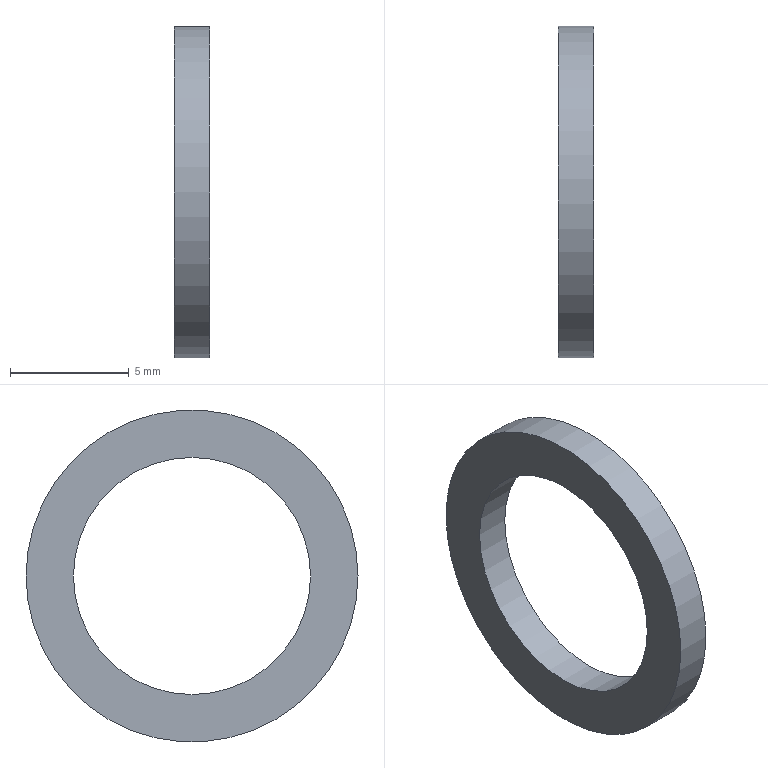Component | NX | TUBE_SEAL | 1 solid | 4 faces | box 1.5 x 14 x 14 mm | volume 113 mm3 | cylinder 2 | plane 2 | commonest cylinder face diameters 14 x1 10 x1
STEP:
#1=CARTESIAN_POINT('',(0.,0.,0.));
#2=DIRECTION('',(0.,0.,1.));
#3=DIRECTION('',(1.,0.,0.));
#4=AXIS2_PLACEMENT_3D('',#1,#2,#3);
#5=CARTESIAN_POINT('',(50.5,3.5,-140.938));
#6=VERTEX_POINT('',#5);
#7=CARTESIAN_POINT('',(50.5,-0.,-147.));
#8=DIRECTION('',(1.,0.,0.));
#9=DIRECTION('',(0.,0.5,0.866));
#10=AXIS2_PLACEMENT_3D('',#7,#8,#9);
#11=CIRCLE('',#10,7.);
#12=CARTESIAN_POINT('',(50.5,-0.,-147.));
#13=DIRECTION('',(-1.,0.,0.));
#14=DIRECTION('',(0.,-0.5,-0.866));
#15=AXIS2_PLACEMENT_3D('',#12,#13,#14);
#16=CYLINDRICAL_SURFACE('',#15,7.);
#17=CARTESIAN_POINT('',(9.425,0.));
#18=DIRECTION('',(-1.,0.));
#19=VECTOR('',#18,1.);
#20=LINE('',#17,#19);
#21=(GEOMETRIC_REPRESENTATION_CONTEXT(2)PARAMETRIC_REPRESENTATION_CONTEXT()REPRESENTATION_CONTEXT('',''));
#22=DEFINITIONAL_REPRESENTATION('',(#20),#21);
#23=PCURVE('',#16,#22);
#24=CARTESIAN_POINT('',(50.5,-0.,-147.));
#25=DIRECTION('',(1.,0.,0.));
#26=DIRECTION('',(0.,0.5,0.866));
#27=AXIS2_PLACEMENT_3D('',#24,#25,#26);
#28=PLANE('',#27);
#29=CARTESIAN_POINT('',(0.,0.));
#30=DIRECTION('',(1.,0.));
#31=AXIS2_PLACEMENT_2D('',#29,#30);
#32=CIRCLE('',#31,7.);
#33=(GEOMETRIC_REPRESENTATION_CONTEXT(2)PARAMETRIC_REPRESENTATION_CONTEXT()REPRESENTATION_CONTEXT('',''));
#34=DEFINITIONAL_REPRESENTATION('',(#32),#33);
#35=PCURVE('',#28,#34);
#36=SURFACE_CURVE('',#11,(#23,#35),.PCURVE_S1.);
#37=EDGE_CURVE('',#6,#6,#36,.T.);
#38=ORIENTED_EDGE('',*,*,#37,.F.);
#39=CARTESIAN_POINT('',(49.,3.5,-140.938));
#40=VERTEX_POINT('',#39);
#41=CARTESIAN_POINT('',(50.5,3.5,-140.938));
#42=CARTESIAN_POINT('',(49.,3.5,-140.938));
#43=B_SPLINE_CURVE_WITH_KNOTS('',1,(#41,#42),.UNSPECIFIED.,.F.,.F.,(2,2),(0.,1.5),.PIECEWISE_BEZIER_KNOTS.);
#44=CARTESIAN_POINT('',(9.425,0.));
#45=DIRECTION('',(0.,1.));
#46=VECTOR('',#45,1.);
#47=LINE('',#44,#46);
#48=(GEOMETRIC_REPRESENTATION_CONTEXT(2)PARAMETRIC_REPRESENTATION_CONTEXT()REPRESENTATION_CONTEXT('',''));
#49=DEFINITIONAL_REPRESENTATION('',(#47),#48);
#50=PCURVE('',#16,#49);
#51=CARTESIAN_POINT('',(3.142,0.));
#52=DIRECTION('',(0.,1.));
#53=VECTOR('',#52,1.);
#54=LINE('',#51,#53);
#55=(GEOMETRIC_REPRESENTATION_CONTEXT(2)PARAMETRIC_REPRESENTATION_CONTEXT()REPRESENTATION_CONTEXT('',''));
#56=DEFINITIONAL_REPRESENTATION('',(#54),#55);
#57=PCURVE('',#16,#56);
#58=SEAM_CURVE('',#43,(#50,#57),.PCURVE_S1.);
#59=EDGE_CURVE('',#6,#40,#58,.T.);
#60=ORIENTED_EDGE('',*,*,#59,.T.);
#61=CARTESIAN_POINT('',(49.,-0.,-147.));
#62=DIRECTION('',(1.,0.,0.));
#63=DIRECTION('',(0.,0.5,0.866));
#64=AXIS2_PLACEMENT_3D('',#61,#62,#63);
#65=CIRCLE('',#64,7.);
#66=CARTESIAN_POINT('',(9.425,1.5));
#67=DIRECTION('',(-1.,0.));
#68=VECTOR('',#67,1.);
#69=LINE('',#66,#68);
#70=(GEOMETRIC_REPRESENTATION_CONTEXT(2)PARAMETRIC_REPRESENTATION_CONTEXT()REPRESENTATION_CONTEXT('',''));
#71=DEFINITIONAL_REPRESENTATION('',(#69),#70);
#72=PCURVE('',#16,#71);
#73=CARTESIAN_POINT('',(49.,-0.,-147.));
#74=DIRECTION('',(1.,0.,0.));
#75=DIRECTION('',(0.,0.5,0.866));
#76=AXIS2_PLACEMENT_3D('',#73,#74,#75);
#77=PLANE('',#76);
#78=CARTESIAN_POINT('',(0.,0.));
#79=DIRECTION('',(1.,0.));
#80=AXIS2_PLACEMENT_2D('',#78,#79);
#81=CIRCLE('',#80,7.);
#82=(GEOMETRIC_REPRESENTATION_CONTEXT(2)PARAMETRIC_REPRESENTATION_CONTEXT()REPRESENTATION_CONTEXT('',''));
#83=DEFINITIONAL_REPRESENTATION('',(#81),#82);
#84=PCURVE('',#77,#83);
#85=SURFACE_CURVE('',#65,(#72,#84),.PCURVE_S1.);
#86=EDGE_CURVE('',#40,#40,#85,.T.);
#87=ORIENTED_EDGE('',*,*,#86,.T.);
#88=ORIENTED_EDGE('',*,*,#59,.F.);
#89=EDGE_LOOP('',(#38,#60,#87,#88));
#90=FACE_BOUND('',#89,.T.);
#91=ADVANCED_FACE('',(#90),#16,.T.);
#92=CARTESIAN_POINT('',(50.5,2.5,-142.67));
#93=VERTEX_POINT('',#92);
#94=CARTESIAN_POINT('',(50.5,-0.,-147.));
#95=DIRECTION('',(1.,0.,0.));
#96=DIRECTION('',(0.,0.5,0.866));
#97=AXIS2_PLACEMENT_3D('',#94,#95,#96);
#98=CIRCLE('',#97,5.);
#99=CARTESIAN_POINT('',(50.5,-0.,-147.));
#100=DIRECTION('',(-1.,0.,0.));
#101=DIRECTION('',(0.,-0.5,-0.866));
#102=AXIS2_PLACEMENT_3D('',#99,#100,#101);
#103=CYLINDRICAL_SURFACE('',#102,5.);
#104=CARTESIAN_POINT('',(9.425,0.));
#105=DIRECTION('',(-1.,0.));
#106=VECTOR('',#105,1.);
#107=LINE('',#104,#106);
#108=(GEOMETRIC_REPRESENTATION_CONTEXT(2)PARAMETRIC_REPRESENTATION_CONTEXT()REPRESENTATION_CONTEXT('',''));
#109=DEFINITIONAL_REPRESENTATION('',(#107),#108);
#110=PCURVE('',#103,#109);
#111=CARTESIAN_POINT('',(0.,0.));
#112=DIRECTION('',(1.,-0.));
#113=AXIS2_PLACEMENT_2D('',#111,#112);
#114=CIRCLE('',#113,5.);
#115=(GEOMETRIC_REPRESENTATION_CONTEXT(2)PARAMETRIC_REPRESENTATION_CONTEXT()REPRESENTATION_CONTEXT('',''));
#116=DEFINITIONAL_REPRESENTATION('',(#114),#115);
#117=PCURVE('',#28,#116);
#118=SURFACE_CURVE('',#98,(#110,#117),.PCURVE_S1.);
#119=EDGE_CURVE('',#93,#93,#118,.T.);
#120=ORIENTED_EDGE('',*,*,#119,.F.);
#121=CARTESIAN_POINT('',(49.,2.5,-142.67));
#122=VERTEX_POINT('',#121);
#123=CARTESIAN_POINT('',(50.5,2.5,-142.67));
#124=CARTESIAN_POINT('',(49.,2.5,-142.67));
#125=B_SPLINE_CURVE_WITH_KNOTS('',1,(#123,#124),.UNSPECIFIED.,.F.,.F.,(2,2),(0.,1.5),.PIECEWISE_BEZIER_KNOTS.);
#126=CARTESIAN_POINT('',(9.425,0.));
#127=DIRECTION('',(0.,1.));
#128=VECTOR('',#127,1.);
#129=LINE('',#126,#128);
#130=(GEOMETRIC_REPRESENTATION_CONTEXT(2)PARAMETRIC_REPRESENTATION_CONTEXT()REPRESENTATION_CONTEXT('',''));
#131=DEFINITIONAL_REPRESENTATION('',(#129),#130);
#132=PCURVE('',#103,#131);
#133=CARTESIAN_POINT('',(3.142,0.));
#134=DIRECTION('',(0.,1.));
#135=VECTOR('',#134,1.);
#136=LINE('',#133,#135);
#137=(GEOMETRIC_REPRESENTATION_CONTEXT(2)PARAMETRIC_REPRESENTATION_CONTEXT()REPRESENTATION_CONTEXT('',''));
#138=DEFINITIONAL_REPRESENTATION('',(#136),#137);
#139=PCURVE('',#103,#138);
#140=SEAM_CURVE('',#125,(#132,#139),.PCURVE_S1.);
#141=EDGE_CURVE('',#93,#122,#140,.T.);
#142=ORIENTED_EDGE('',*,*,#141,.T.);
#143=CARTESIAN_POINT('',(49.,-0.,-147.));
#144=DIRECTION('',(1.,0.,0.));
#145=DIRECTION('',(0.,0.5,0.866));
#146=AXIS2_PLACEMENT_3D('',#143,#144,#145);
#147=CIRCLE('',#146,5.);
#148=CARTESIAN_POINT('',(9.425,1.5));
#149=DIRECTION('',(-1.,0.));
#150=VECTOR('',#149,1.);
#151=LINE('',#148,#150);
#152=(GEOMETRIC_REPRESENTATION_CONTEXT(2)PARAMETRIC_REPRESENTATION_CONTEXT()REPRESENTATION_CONTEXT('',''));
#153=DEFINITIONAL_REPRESENTATION('',(#151),#152);
#154=PCURVE('',#103,#153);
#155=CARTESIAN_POINT('',(0.,0.));
#156=DIRECTION('',(1.,-0.));
#157=AXIS2_PLACEMENT_2D('',#155,#156);
#158=CIRCLE('',#157,5.);
#159=(GEOMETRIC_REPRESENTATION_CONTEXT(2)PARAMETRIC_REPRESENTATION_CONTEXT()REPRESENTATION_CONTEXT('',''));
#160=DEFINITIONAL_REPRESENTATION('',(#158),#159);
#161=PCURVE('',#77,#160);
#162=SURFACE_CURVE('',#147,(#154,#161),.PCURVE_S1.);
#163=EDGE_CURVE('',#122,#122,#162,.T.);
#164=ORIENTED_EDGE('',*,*,#163,.T.);
#165=ORIENTED_EDGE('',*,*,#141,.F.);
#166=EDGE_LOOP('',(#120,#142,#164,#165));
#167=FACE_BOUND('',#166,.F.);
#168=ADVANCED_FACE('',(#167),#103,.F.);
#169=ORIENTED_EDGE('',*,*,#37,.T.);
#170=EDGE_LOOP('',(#169));
#171=FACE_BOUND('',#170,.T.);
#172=ORIENTED_EDGE('',*,*,#119,.F.);
#173=EDGE_LOOP('',(#172));
#174=FACE_BOUND('',#173,.T.);
#175=ADVANCED_FACE('',(#171,#174),#28,.T.);
#176=ORIENTED_EDGE('',*,*,#86,.F.);
#177=EDGE_LOOP('',(#176));
#178=FACE_BOUND('',#177,.T.);
#179=ORIENTED_EDGE('',*,*,#163,.T.);
#180=EDGE_LOOP('',(#179));
#181=FACE_BOUND('',#180,.T.);
#182=ADVANCED_FACE('',(#178,#181),#77,.F.);
#183=CLOSED_SHELL('',(#91,#168,#175,#182));
#184=MANIFOLD_SOLID_BREP('',#183);
#185=(LENGTH_UNIT()NAMED_UNIT(*)SI_UNIT(.MILLI.,.METRE.));
#186=UNCERTAINTY_MEASURE_WITH_UNIT(LENGTH_MEASURE(0.00001),#185,'','');
#187=(NAMED_UNIT(*)PLANE_ANGLE_UNIT()SI_UNIT($,.RADIAN.));
#188=(NAMED_UNIT(*)SI_UNIT($,.STERADIAN.)SOLID_ANGLE_UNIT());
#189=(GEOMETRIC_REPRESENTATION_CONTEXT(3)GLOBAL_UNCERTAINTY_ASSIGNED_CONTEXT((#186))GLOBAL_UNIT_ASSIGNED_CONTEXT((#185,#187,#188))REPRESENTATION_CONTEXT('',''));
#190=ADVANCED_BREP_SHAPE_REPRESENTATION('',(#4,#184),#189);